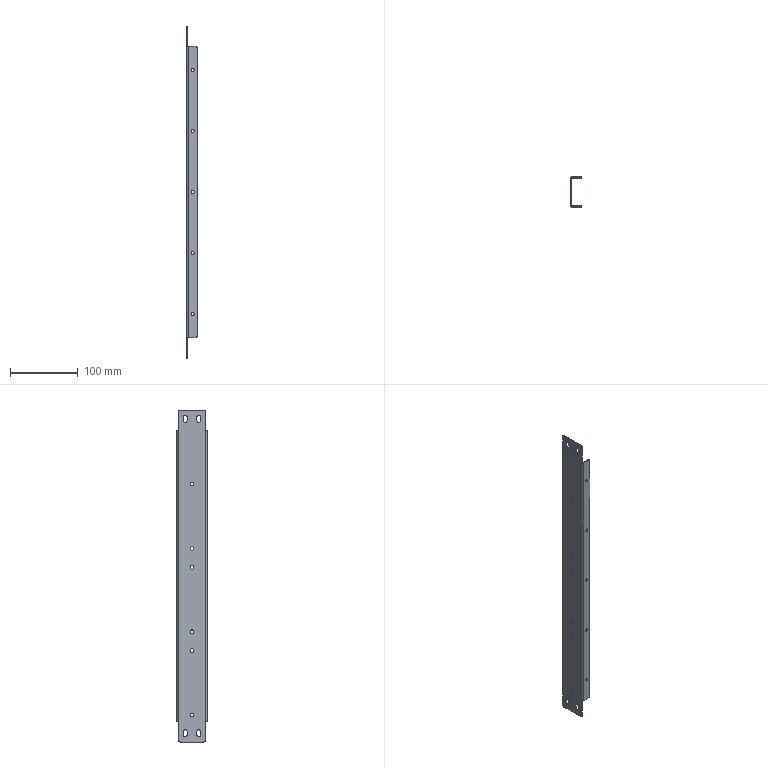Component | SolidWorks | CompositeSwitchMountingBeam100-7 | 1 solid | 86 faces | volume 48147 mm3 | cylinder 56 | plane 30 | commonest cylinder face diameters 5.5 x24 4.5 x20 6 x8 4.473 x2 1.473 x2